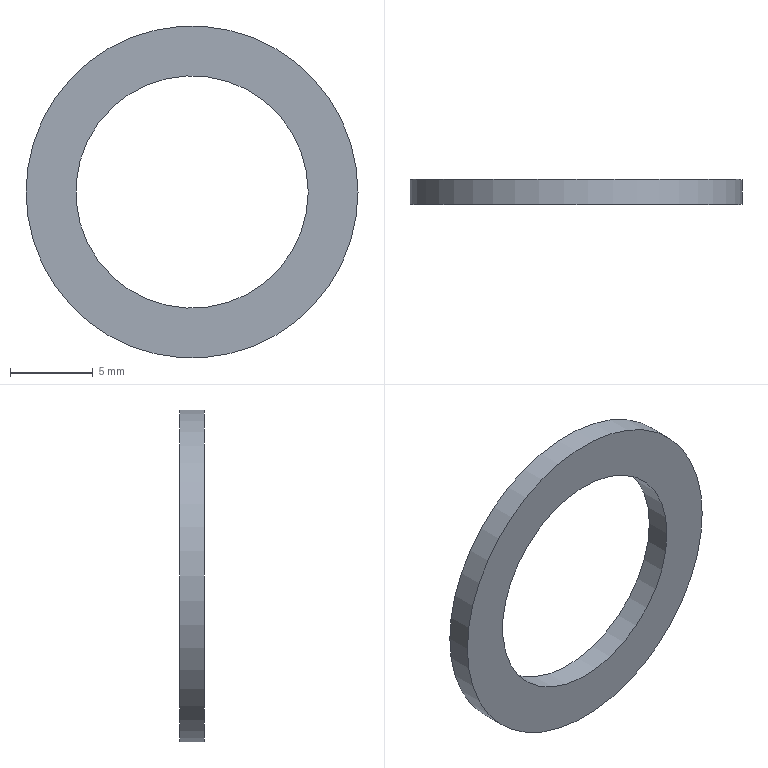Component | NX | LARGE_WASHER | 1 solid | 4 faces | box 20 x 1.5 x 20 mm | volume 240 mm3 | cylinder 2 | plane 2 | commonest cylinder face diameters 20 x1 14 x1
STEP:
#1=CARTESIAN_POINT('',(0.,0.,0.));
#2=DIRECTION('',(0.,0.,1.));
#3=DIRECTION('',(1.,0.,0.));
#4=AXIS2_PLACEMENT_3D('',#1,#2,#3);
#5=CARTESIAN_POINT('',(23.994,-126.616,-0.));
#6=VERTEX_POINT('',#5);
#7=CARTESIAN_POINT('',(13.994,-126.616,-0.));
#8=DIRECTION('',(0.,-1.,0.));
#9=DIRECTION('',(1.,0.,-0.));
#10=AXIS2_PLACEMENT_3D('',#7,#8,#9);
#11=CIRCLE('',#10,10.);
#12=CARTESIAN_POINT('',(13.994,-126.616,-0.));
#13=DIRECTION('',(0.,1.,0.));
#14=DIRECTION('',(0.,0.,1.));
#15=AXIS2_PLACEMENT_3D('',#12,#13,#14);
#16=CYLINDRICAL_SURFACE('',#15,10.);
#17=CARTESIAN_POINT('',(7.854,0.));
#18=DIRECTION('',(-1.,0.));
#19=VECTOR('',#18,1.);
#20=LINE('',#17,#19);
#21=(GEOMETRIC_REPRESENTATION_CONTEXT(2)PARAMETRIC_REPRESENTATION_CONTEXT()REPRESENTATION_CONTEXT('',''));
#22=DEFINITIONAL_REPRESENTATION('',(#20),#21);
#23=PCURVE('',#16,#22);
#24=CARTESIAN_POINT('',(13.994,-126.616,-0.));
#25=DIRECTION('',(0.,-1.,0.));
#26=DIRECTION('',(0.,0.,-1.));
#27=AXIS2_PLACEMENT_3D('',#24,#25,#26);
#28=PLANE('',#27);
#29=CARTESIAN_POINT('',(0.,0.));
#30=DIRECTION('',(0.,1.));
#31=AXIS2_PLACEMENT_2D('',#29,#30);
#32=CIRCLE('',#31,10.);
#33=(GEOMETRIC_REPRESENTATION_CONTEXT(2)PARAMETRIC_REPRESENTATION_CONTEXT()REPRESENTATION_CONTEXT('',''));
#34=DEFINITIONAL_REPRESENTATION('',(#32),#33);
#35=PCURVE('',#28,#34);
#36=SURFACE_CURVE('',#11,(#23,#35),.PCURVE_S1.);
#37=EDGE_CURVE('',#6,#6,#36,.T.);
#38=ORIENTED_EDGE('',*,*,#37,.F.);
#39=CARTESIAN_POINT('',(23.994,-125.116,-0.));
#40=VERTEX_POINT('',#39);
#41=CARTESIAN_POINT('',(23.994,-126.616,-0.));
#42=CARTESIAN_POINT('',(23.994,-125.116,-0.));
#43=B_SPLINE_CURVE_WITH_KNOTS('',1,(#41,#42),.UNSPECIFIED.,.F.,.F.,(2,2),(0.,1.5),.PIECEWISE_BEZIER_KNOTS.);
#44=CARTESIAN_POINT('',(7.854,0.));
#45=DIRECTION('',(0.,1.));
#46=VECTOR('',#45,1.);
#47=LINE('',#44,#46);
#48=(GEOMETRIC_REPRESENTATION_CONTEXT(2)PARAMETRIC_REPRESENTATION_CONTEXT()REPRESENTATION_CONTEXT('',''));
#49=DEFINITIONAL_REPRESENTATION('',(#47),#48);
#50=PCURVE('',#16,#49);
#51=CARTESIAN_POINT('',(1.571,0.));
#52=DIRECTION('',(0.,1.));
#53=VECTOR('',#52,1.);
#54=LINE('',#51,#53);
#55=(GEOMETRIC_REPRESENTATION_CONTEXT(2)PARAMETRIC_REPRESENTATION_CONTEXT()REPRESENTATION_CONTEXT('',''));
#56=DEFINITIONAL_REPRESENTATION('',(#54),#55);
#57=PCURVE('',#16,#56);
#58=SEAM_CURVE('',#43,(#50,#57),.PCURVE_S1.);
#59=EDGE_CURVE('',#6,#40,#58,.T.);
#60=ORIENTED_EDGE('',*,*,#59,.T.);
#61=CARTESIAN_POINT('',(13.994,-125.116,-0.));
#62=DIRECTION('',(0.,-1.,0.));
#63=DIRECTION('',(1.,0.,-0.));
#64=AXIS2_PLACEMENT_3D('',#61,#62,#63);
#65=CIRCLE('',#64,10.);
#66=CARTESIAN_POINT('',(7.854,1.5));
#67=DIRECTION('',(-1.,0.));
#68=VECTOR('',#67,1.);
#69=LINE('',#66,#68);
#70=(GEOMETRIC_REPRESENTATION_CONTEXT(2)PARAMETRIC_REPRESENTATION_CONTEXT()REPRESENTATION_CONTEXT('',''));
#71=DEFINITIONAL_REPRESENTATION('',(#69),#70);
#72=PCURVE('',#16,#71);
#73=CARTESIAN_POINT('',(13.994,-125.116,-0.));
#74=DIRECTION('',(0.,-1.,0.));
#75=DIRECTION('',(0.,0.,-1.));
#76=AXIS2_PLACEMENT_3D('',#73,#74,#75);
#77=PLANE('',#76);
#78=CARTESIAN_POINT('',(0.,0.));
#79=DIRECTION('',(0.,1.));
#80=AXIS2_PLACEMENT_2D('',#78,#79);
#81=CIRCLE('',#80,10.);
#82=(GEOMETRIC_REPRESENTATION_CONTEXT(2)PARAMETRIC_REPRESENTATION_CONTEXT()REPRESENTATION_CONTEXT('',''));
#83=DEFINITIONAL_REPRESENTATION('',(#81),#82);
#84=PCURVE('',#77,#83);
#85=SURFACE_CURVE('',#65,(#72,#84),.PCURVE_S1.);
#86=EDGE_CURVE('',#40,#40,#85,.T.);
#87=ORIENTED_EDGE('',*,*,#86,.T.);
#88=ORIENTED_EDGE('',*,*,#59,.F.);
#89=EDGE_LOOP('',(#38,#60,#87,#88));
#90=FACE_BOUND('',#89,.T.);
#91=ADVANCED_FACE('',(#90),#16,.T.);
#92=CARTESIAN_POINT('',(20.994,-126.616,-0.));
#93=VERTEX_POINT('',#92);
#94=CARTESIAN_POINT('',(13.994,-126.616,-0.));
#95=DIRECTION('',(0.,-1.,0.));
#96=DIRECTION('',(1.,0.,-0.));
#97=AXIS2_PLACEMENT_3D('',#94,#95,#96);
#98=CIRCLE('',#97,7.);
#99=CARTESIAN_POINT('',(13.994,-126.616,-0.));
#100=DIRECTION('',(0.,1.,0.));
#101=DIRECTION('',(0.,0.,1.));
#102=AXIS2_PLACEMENT_3D('',#99,#100,#101);
#103=CYLINDRICAL_SURFACE('',#102,7.);
#104=CARTESIAN_POINT('',(7.854,0.));
#105=DIRECTION('',(-1.,0.));
#106=VECTOR('',#105,1.);
#107=LINE('',#104,#106);
#108=(GEOMETRIC_REPRESENTATION_CONTEXT(2)PARAMETRIC_REPRESENTATION_CONTEXT()REPRESENTATION_CONTEXT('',''));
#109=DEFINITIONAL_REPRESENTATION('',(#107),#108);
#110=PCURVE('',#103,#109);
#111=CARTESIAN_POINT('',(0.,0.));
#112=DIRECTION('',(0.,1.));
#113=AXIS2_PLACEMENT_2D('',#111,#112);
#114=CIRCLE('',#113,7.);
#115=(GEOMETRIC_REPRESENTATION_CONTEXT(2)PARAMETRIC_REPRESENTATION_CONTEXT()REPRESENTATION_CONTEXT('',''));
#116=DEFINITIONAL_REPRESENTATION('',(#114),#115);
#117=PCURVE('',#28,#116);
#118=SURFACE_CURVE('',#98,(#110,#117),.PCURVE_S1.);
#119=EDGE_CURVE('',#93,#93,#118,.T.);
#120=ORIENTED_EDGE('',*,*,#119,.F.);
#121=CARTESIAN_POINT('',(20.994,-125.116,-0.));
#122=VERTEX_POINT('',#121);
#123=CARTESIAN_POINT('',(20.994,-126.616,-0.));
#124=CARTESIAN_POINT('',(20.994,-125.116,-0.));
#125=B_SPLINE_CURVE_WITH_KNOTS('',1,(#123,#124),.UNSPECIFIED.,.F.,.F.,(2,2),(0.,1.5),.PIECEWISE_BEZIER_KNOTS.);
#126=CARTESIAN_POINT('',(7.854,0.));
#127=DIRECTION('',(0.,1.));
#128=VECTOR('',#127,1.);
#129=LINE('',#126,#128);
#130=(GEOMETRIC_REPRESENTATION_CONTEXT(2)PARAMETRIC_REPRESENTATION_CONTEXT()REPRESENTATION_CONTEXT('',''));
#131=DEFINITIONAL_REPRESENTATION('',(#129),#130);
#132=PCURVE('',#103,#131);
#133=CARTESIAN_POINT('',(1.571,0.));
#134=DIRECTION('',(0.,1.));
#135=VECTOR('',#134,1.);
#136=LINE('',#133,#135);
#137=(GEOMETRIC_REPRESENTATION_CONTEXT(2)PARAMETRIC_REPRESENTATION_CONTEXT()REPRESENTATION_CONTEXT('',''));
#138=DEFINITIONAL_REPRESENTATION('',(#136),#137);
#139=PCURVE('',#103,#138);
#140=SEAM_CURVE('',#125,(#132,#139),.PCURVE_S1.);
#141=EDGE_CURVE('',#93,#122,#140,.T.);
#142=ORIENTED_EDGE('',*,*,#141,.T.);
#143=CARTESIAN_POINT('',(13.994,-125.116,-0.));
#144=DIRECTION('',(0.,-1.,0.));
#145=DIRECTION('',(1.,0.,-0.));
#146=AXIS2_PLACEMENT_3D('',#143,#144,#145);
#147=CIRCLE('',#146,7.);
#148=CARTESIAN_POINT('',(7.854,1.5));
#149=DIRECTION('',(-1.,0.));
#150=VECTOR('',#149,1.);
#151=LINE('',#148,#150);
#152=(GEOMETRIC_REPRESENTATION_CONTEXT(2)PARAMETRIC_REPRESENTATION_CONTEXT()REPRESENTATION_CONTEXT('',''));
#153=DEFINITIONAL_REPRESENTATION('',(#151),#152);
#154=PCURVE('',#103,#153);
#155=CARTESIAN_POINT('',(0.,0.));
#156=DIRECTION('',(0.,1.));
#157=AXIS2_PLACEMENT_2D('',#155,#156);
#158=CIRCLE('',#157,7.);
#159=(GEOMETRIC_REPRESENTATION_CONTEXT(2)PARAMETRIC_REPRESENTATION_CONTEXT()REPRESENTATION_CONTEXT('',''));
#160=DEFINITIONAL_REPRESENTATION('',(#158),#159);
#161=PCURVE('',#77,#160);
#162=SURFACE_CURVE('',#147,(#154,#161),.PCURVE_S1.);
#163=EDGE_CURVE('',#122,#122,#162,.T.);
#164=ORIENTED_EDGE('',*,*,#163,.T.);
#165=ORIENTED_EDGE('',*,*,#141,.F.);
#166=EDGE_LOOP('',(#120,#142,#164,#165));
#167=FACE_BOUND('',#166,.F.);
#168=ADVANCED_FACE('',(#167),#103,.F.);
#169=ORIENTED_EDGE('',*,*,#37,.T.);
#170=EDGE_LOOP('',(#169));
#171=FACE_BOUND('',#170,.T.);
#172=ORIENTED_EDGE('',*,*,#119,.F.);
#173=EDGE_LOOP('',(#172));
#174=FACE_BOUND('',#173,.T.);
#175=ADVANCED_FACE('',(#171,#174),#28,.T.);
#176=ORIENTED_EDGE('',*,*,#86,.F.);
#177=EDGE_LOOP('',(#176));
#178=FACE_BOUND('',#177,.T.);
#179=ORIENTED_EDGE('',*,*,#163,.T.);
#180=EDGE_LOOP('',(#179));
#181=FACE_BOUND('',#180,.T.);
#182=ADVANCED_FACE('',(#178,#181),#77,.F.);
#183=CLOSED_SHELL('',(#91,#168,#175,#182));
#184=MANIFOLD_SOLID_BREP('',#183);
#185=(LENGTH_UNIT()NAMED_UNIT(*)SI_UNIT(.MILLI.,.METRE.));
#186=UNCERTAINTY_MEASURE_WITH_UNIT(LENGTH_MEASURE(0.00001),#185,'','');
#187=(NAMED_UNIT(*)PLANE_ANGLE_UNIT()SI_UNIT($,.RADIAN.));
#188=(NAMED_UNIT(*)SI_UNIT($,.STERADIAN.)SOLID_ANGLE_UNIT());
#189=(GEOMETRIC_REPRESENTATION_CONTEXT(3)GLOBAL_UNCERTAINTY_ASSIGNED_CONTEXT((#186))GLOBAL_UNIT_ASSIGNED_CONTEXT((#185,#187,#188))REPRESENTATION_CONTEXT('',''));
#190=ADVANCED_BREP_SHAPE_REPRESENTATION('',(#4,#184),#189);